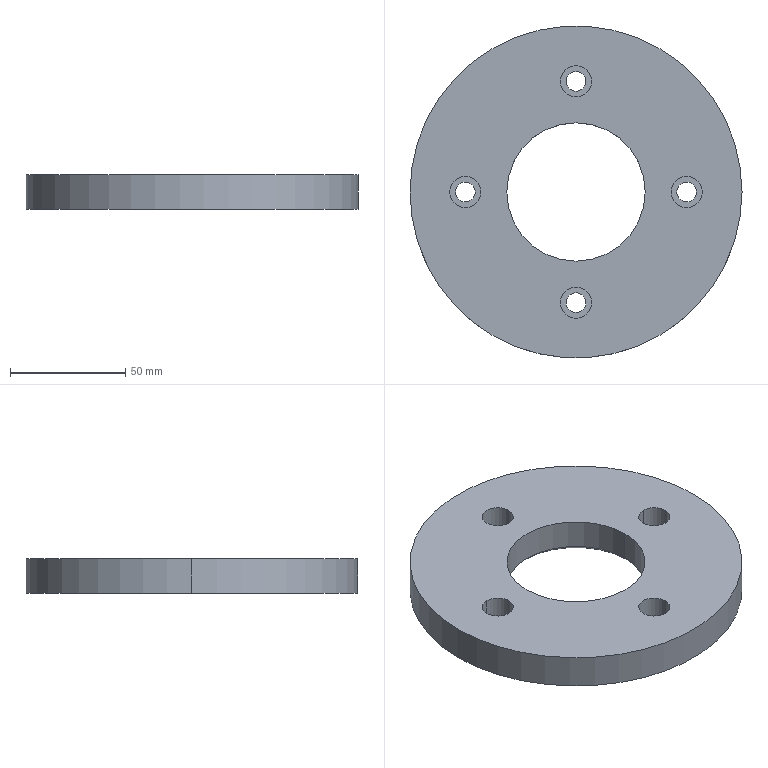CAM job | Mastercam | mm | 14 operations | part box 144 x 144 x 15
1. Facing | 13 - 50 圆鼻铣刀
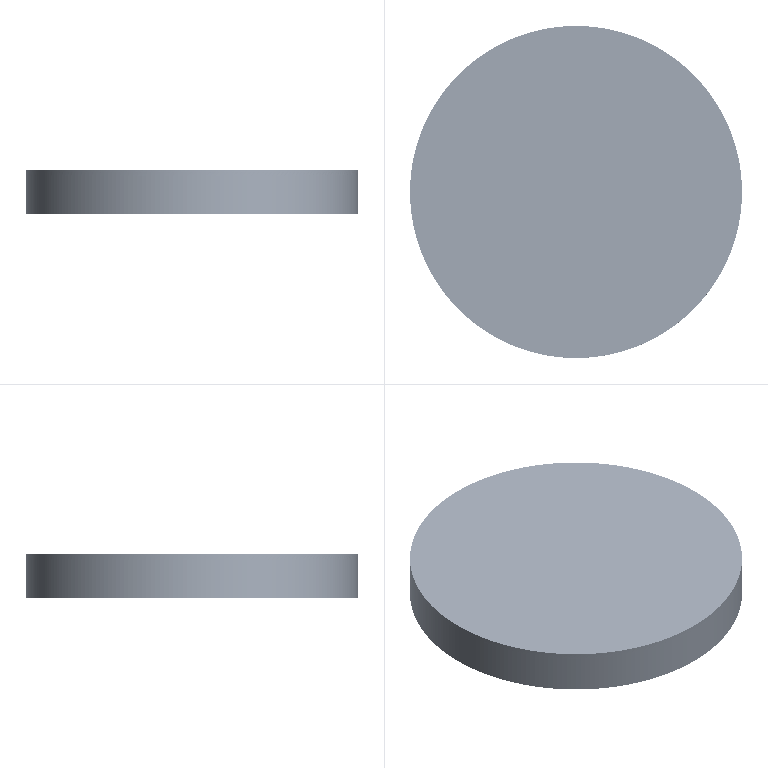2. 2D High Speed (2D Dynamic Mill) | 2 - 12 平铣刀
3. 2D High Speed (2D Dynamic Mill) | 2 - 12 平铣刀
4. Contour (2D) | 3 - 12 平铣刀
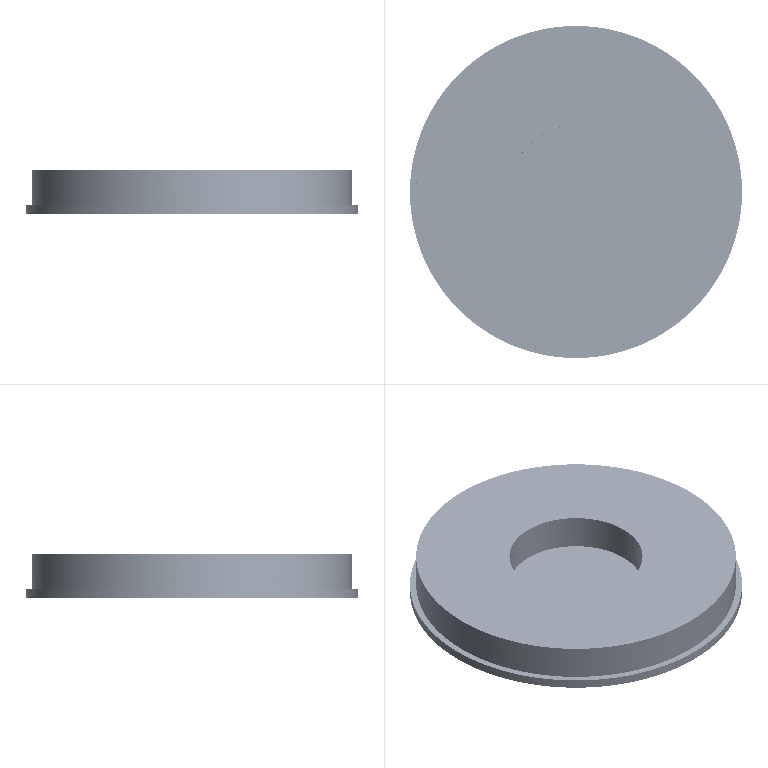5. Contour (2D) | 3 - 12 平铣刀
6. Contour (Ramp) | 4 - 6 平铣刀
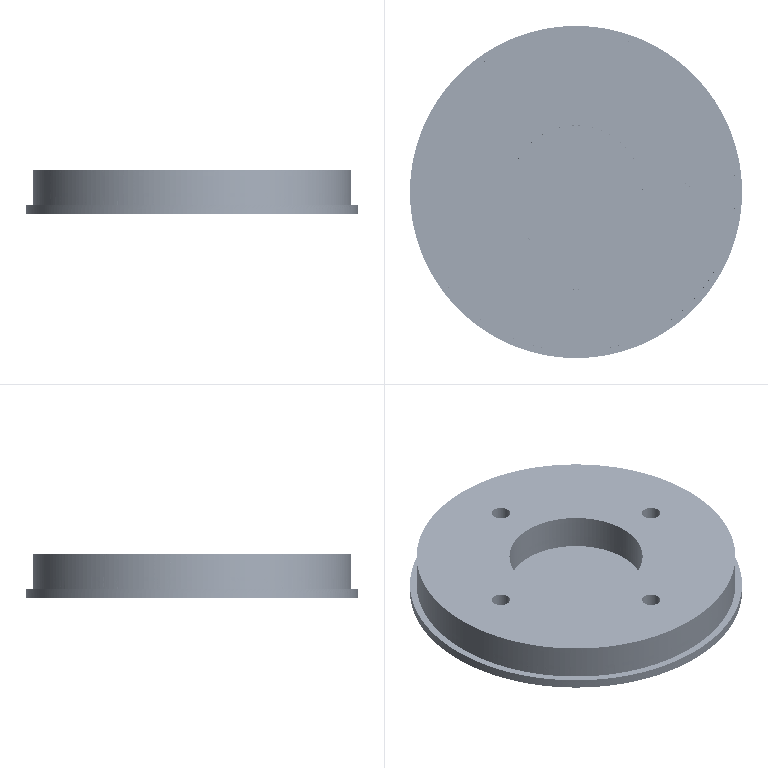7. Contour (Ramp) | 4 - 6 平铣刀
8. Contour (2D) | 5 - 6 平铣刀
9. Contour (2D) | 5 - 6 平铣刀
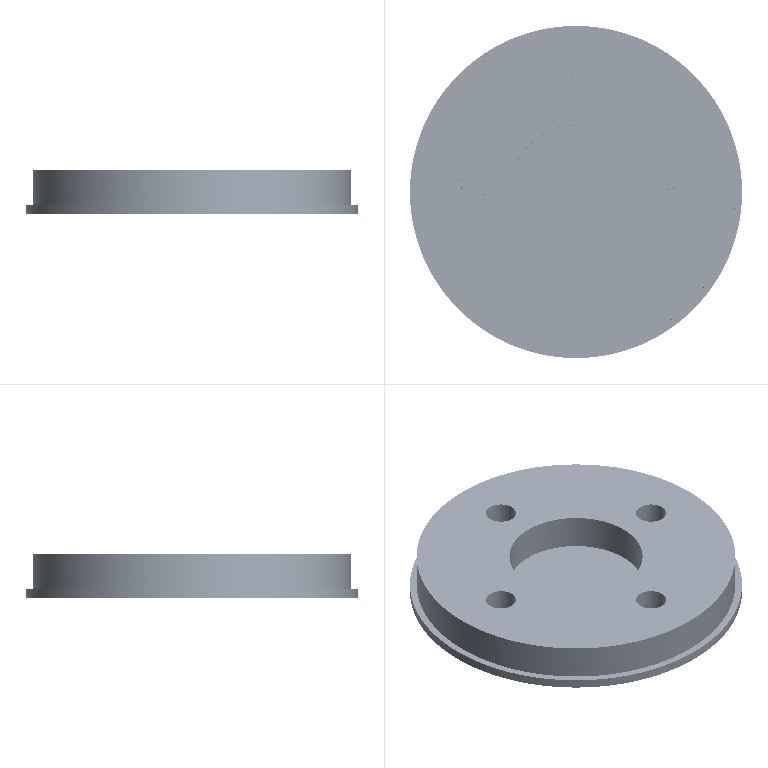10. Model Chamfer | 6 - 6 倒角刀
11. Facing | 13 - 50 圆鼻铣刀
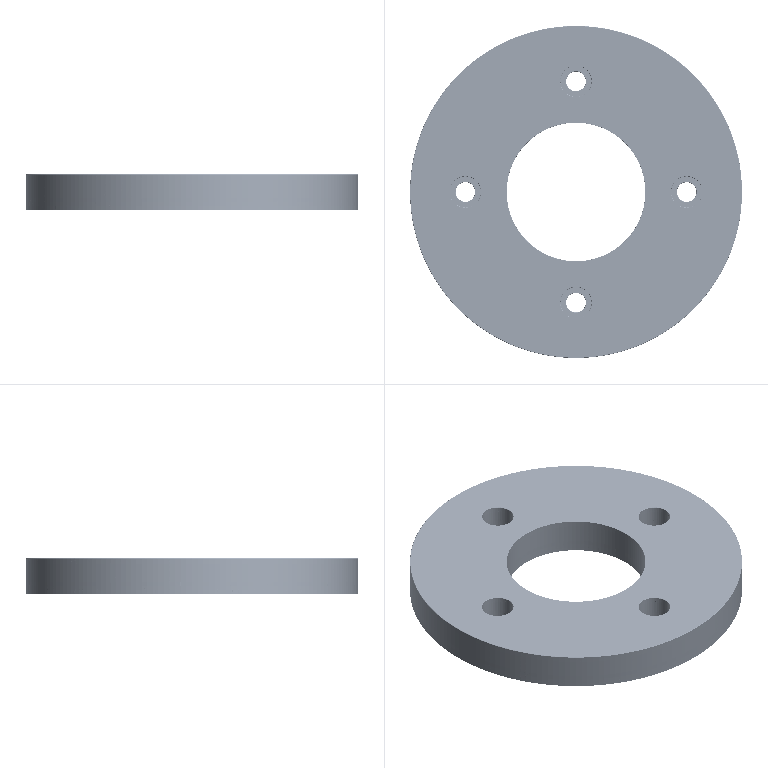12. Facing | 13 - 50 圆鼻铣刀
13. Contour (2D chamfer) | 6 - 6 倒角刀
14. Contour (2D chamfer) | 6 - 6 倒角刀